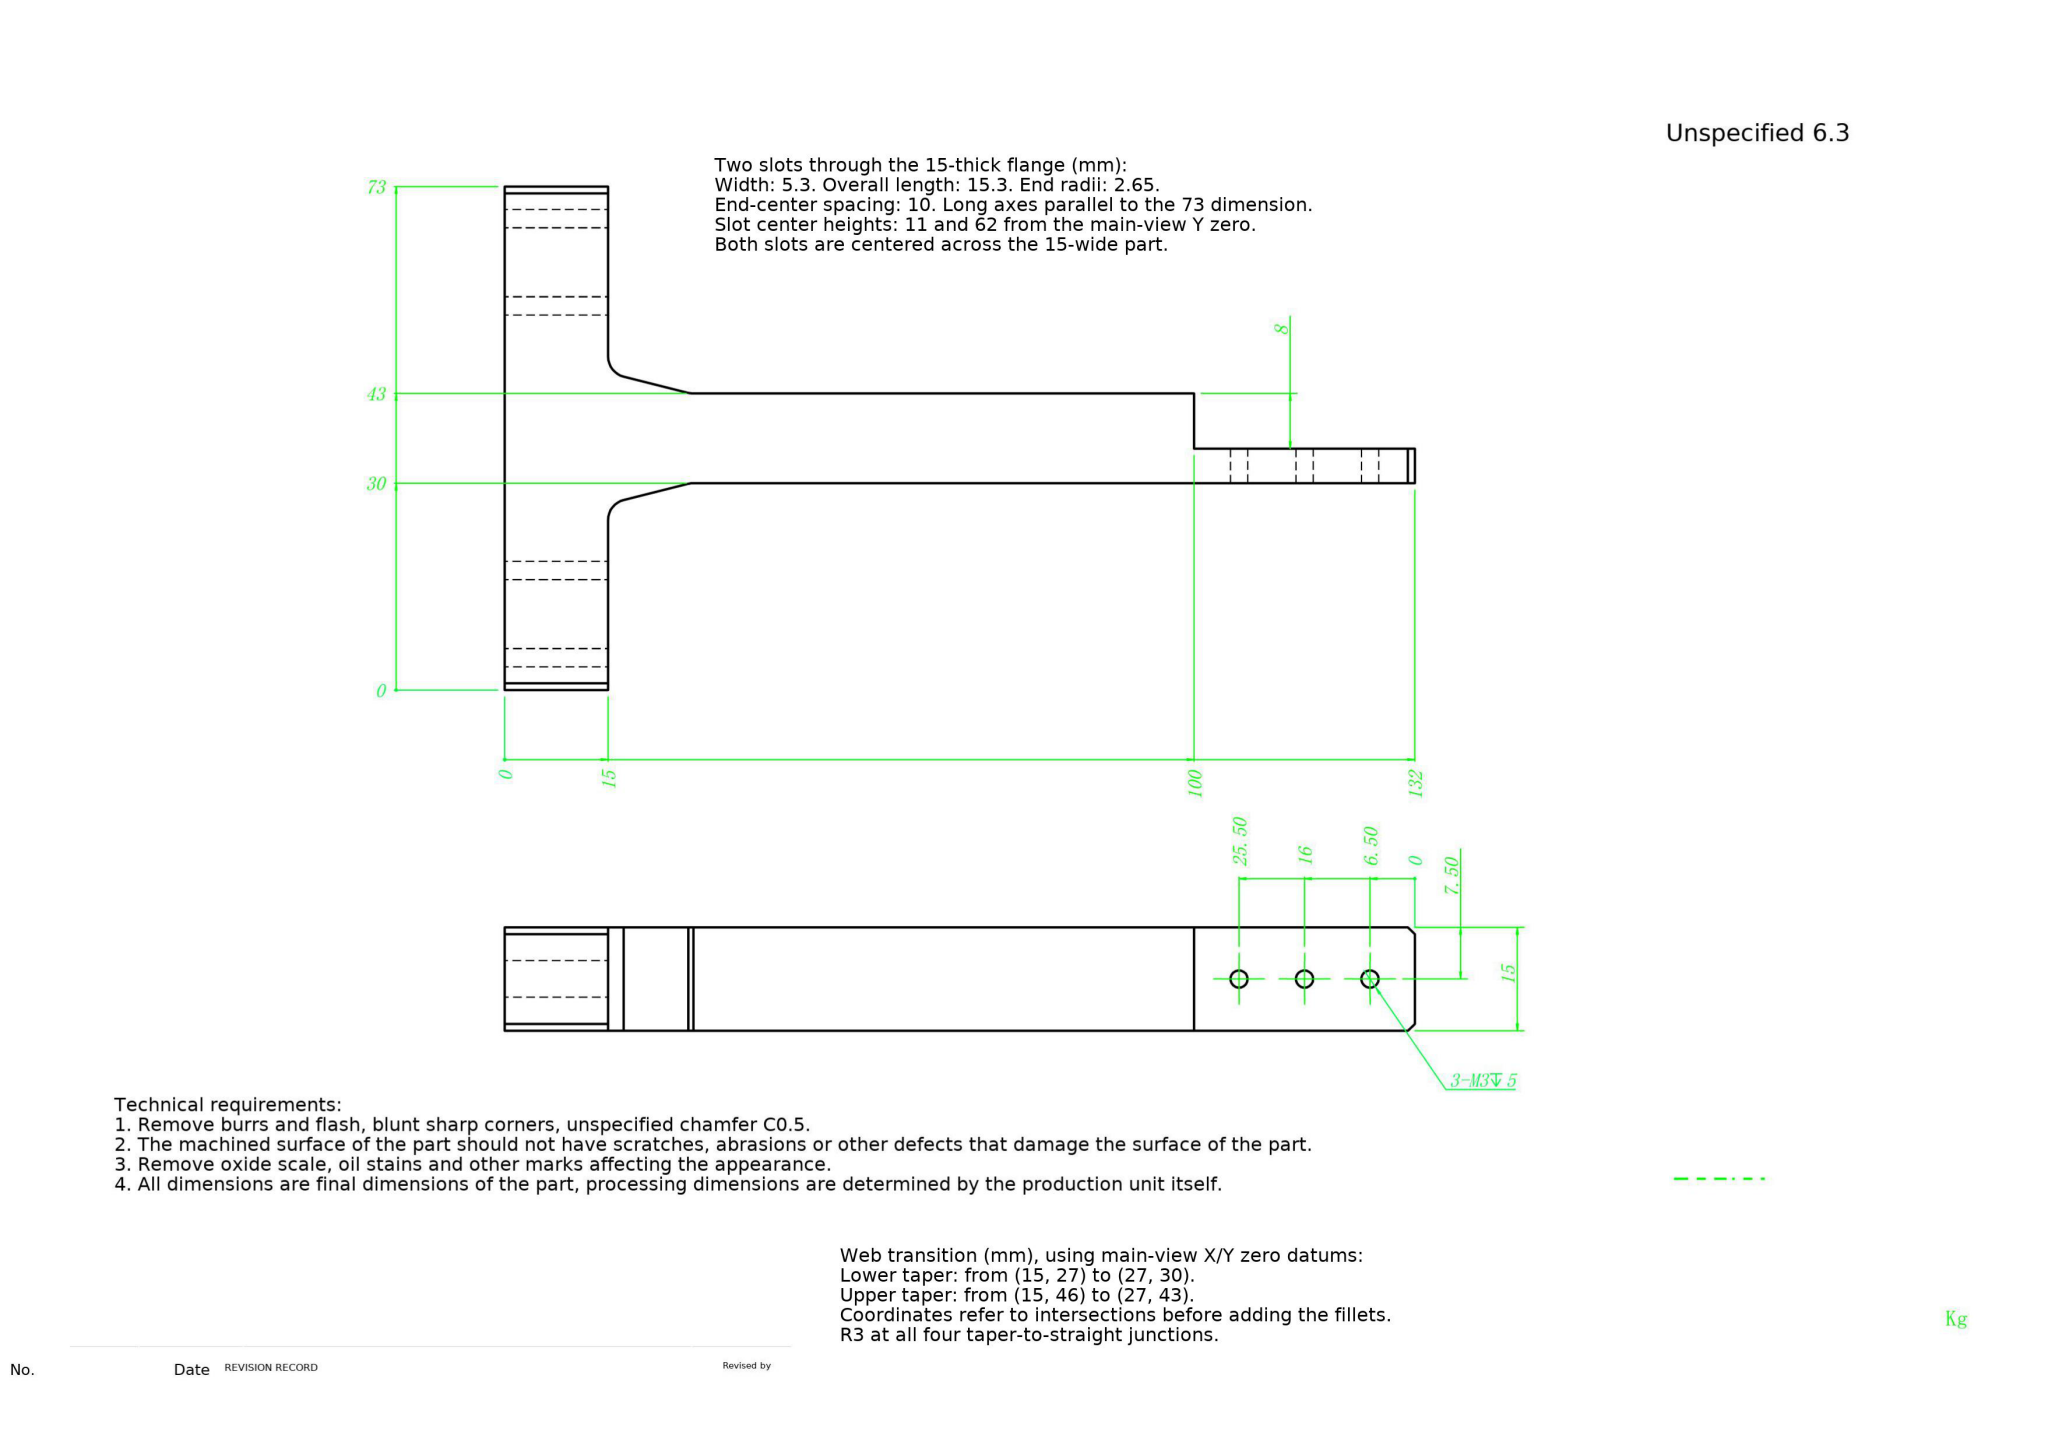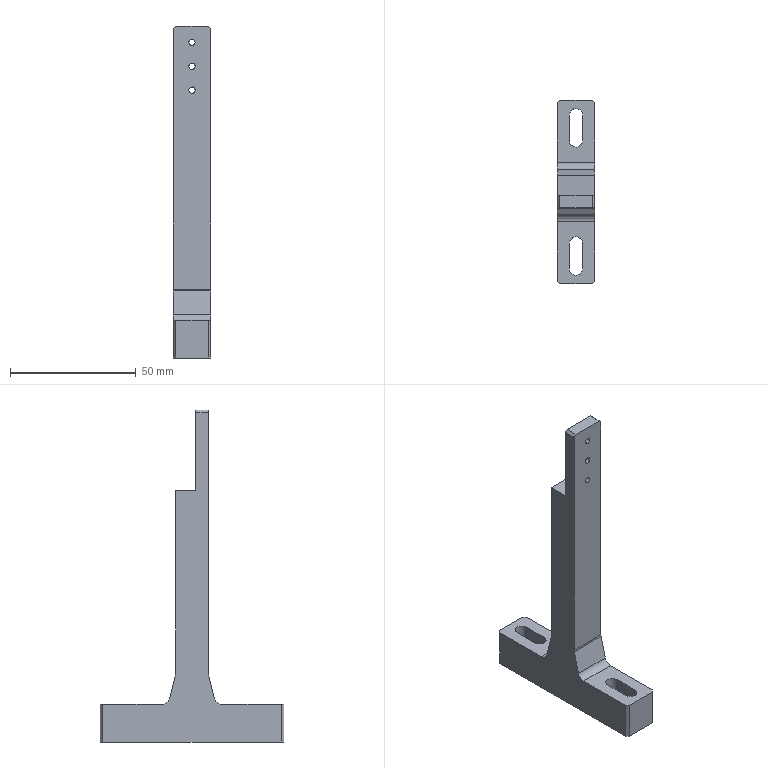Part | NX | mm | Dual-Slot Tall L-Bracket | 1 solid | 38 faces | box 15 x 73 x 132 mm | volume 33612 mm3 | plane 24 | cylinder 14 | commonest cylinder face diameters 2.5 x6 6 x4 5.3 x4